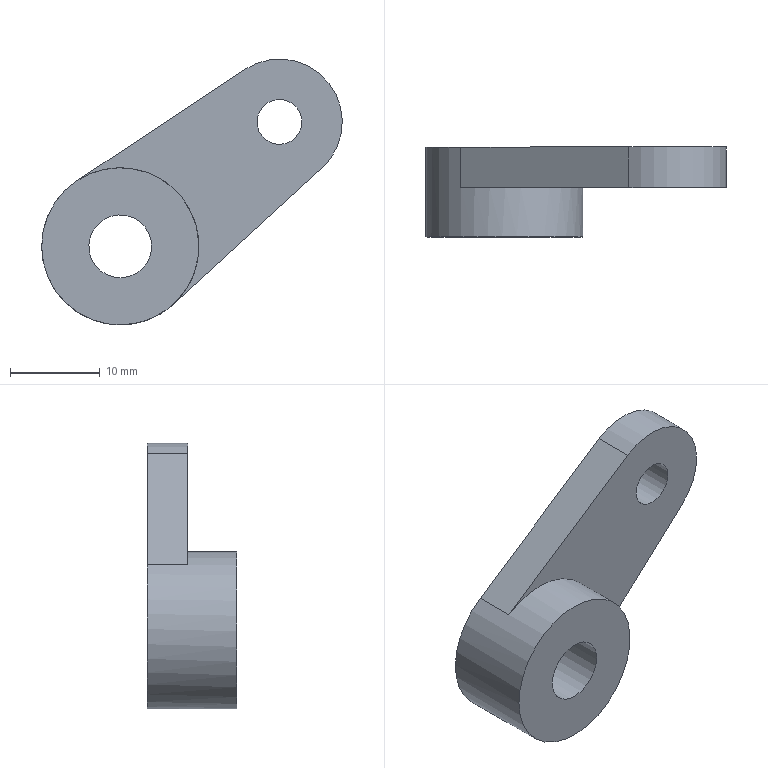Component | NX | 9 | 1 solid | 9 faces | box 33.48 x 10 x 29.6 mm | volume 3337 mm3 | plane 5 | cylinder 4 | commonest cylinder face diameters 14 x1 5 x1 17.5 x1 7 x1
STEP:
#1=CARTESIAN_POINT('',(0.,0.,0.));
#2=DIRECTION('',(0.,0.,1.));
#3=DIRECTION('',(1.,0.,0.));
#4=AXIS2_PLACEMENT_3D('',#1,#2,#3);
#5=CARTESIAN_POINT('',(-294.831,190.749,-231.716));
#6=VERTEX_POINT('',#5);
#7=CARTESIAN_POINT('',(-278.282,190.749,-216.572));
#8=VERTEX_POINT('',#7);
#9=CARTESIAN_POINT('',(-294.831,190.749,-231.716));
#10=DIRECTION('',(0.7377,0.,0.6751));
#11=VECTOR('',#10,1.);
#12=LINE('',#9,#11);
#13=CARTESIAN_POINT('',(-294.831,186.249,-231.716));
#14=DIRECTION('',(-0.6751,0.,0.7377));
#15=DIRECTION('',(-0.7377,0.,-0.6751));
#16=AXIS2_PLACEMENT_3D('',#13,#14,#15);
#17=PLANE('',#16);
#18=CARTESIAN_POINT('',(0.,-4.5));
#19=DIRECTION('',(-1.,0.));
#20=VECTOR('',#19,1.);
#21=LINE('',#18,#20);
#22=(GEOMETRIC_REPRESENTATION_CONTEXT(2)PARAMETRIC_REPRESENTATION_CONTEXT()REPRESENTATION_CONTEXT('',''));
#23=DEFINITIONAL_REPRESENTATION('',(#21),#22);
#24=PCURVE('',#17,#23);
#25=CARTESIAN_POINT('',(-300.738,190.749,-225.261));
#26=DIRECTION('',(0.,1.,0.));
#27=DIRECTION('',(-0.788,0.,-0.6157));
#28=AXIS2_PLACEMENT_3D('',#25,#26,#27);
#29=PLANE('',#28);
#30=CARTESIAN_POINT('',(-0.6806,-8.723));
#31=DIRECTION('',(-0.997,0.07778));
#32=VECTOR('',#31,1.);
#33=LINE('',#30,#32);
#34=(GEOMETRIC_REPRESENTATION_CONTEXT(2)PARAMETRIC_REPRESENTATION_CONTEXT()REPRESENTATION_CONTEXT('',''));
#35=DEFINITIONAL_REPRESENTATION('',(#33),#34);
#36=PCURVE('',#29,#35);
#37=SURFACE_CURVE('',#12,(#24,#36),.PCURVE_S1.);
#38=EDGE_CURVE('',#6,#8,#37,.T.);
#39=ORIENTED_EDGE('',*,*,#38,.T.);
#40=CARTESIAN_POINT('',(-278.282,186.249,-216.572));
#41=VERTEX_POINT('',#40);
#42=CARTESIAN_POINT('',(-278.282,186.249,-216.572));
#43=DIRECTION('',(0.,1.,0.));
#44=VECTOR('',#43,1.);
#45=LINE('',#42,#44);
#46=CARTESIAN_POINT('',(-22.432,0.));
#47=DIRECTION('',(0.,-1.));
#48=VECTOR('',#47,1.);
#49=LINE('',#46,#48);
#50=(GEOMETRIC_REPRESENTATION_CONTEXT(2)PARAMETRIC_REPRESENTATION_CONTEXT()REPRESENTATION_CONTEXT('',''));
#51=DEFINITIONAL_REPRESENTATION('',(#49),#50);
#52=PCURVE('',#17,#51);
#53=CARTESIAN_POINT('',(-283.008,186.249,-211.408));
#54=DIRECTION('',(0.,1.,0.));
#55=DIRECTION('',(-0.788,0.,-0.6157));
#56=AXIS2_PLACEMENT_3D('',#53,#54,#55);
#57=CYLINDRICAL_SURFACE('',#56,7.);
#58=CARTESIAN_POINT('',(4.635,0.));
#59=DIRECTION('',(0.,1.));
#60=VECTOR('',#59,1.);
#61=LINE('',#58,#60);
#62=(GEOMETRIC_REPRESENTATION_CONTEXT(2)PARAMETRIC_REPRESENTATION_CONTEXT()REPRESENTATION_CONTEXT('',''));
#63=DEFINITIONAL_REPRESENTATION('',(#61),#62);
#64=PCURVE('',#57,#63);
#65=SURFACE_CURVE('',#45,(#52,#64),.PCURVE_S1.);
#66=EDGE_CURVE('',#41,#8,#65,.T.);
#67=ORIENTED_EDGE('',*,*,#66,.F.);
#68=CARTESIAN_POINT('',(-294.831,186.249,-231.716));
#69=VERTEX_POINT('',#68);
#70=CARTESIAN_POINT('',(-294.831,186.249,-231.716));
#71=DIRECTION('',(0.7377,0.,0.6751));
#72=VECTOR('',#71,1.);
#73=LINE('',#70,#72);
#74=CARTESIAN_POINT('',(0.,0.));
#75=DIRECTION('',(-1.,0.));
#76=VECTOR('',#75,1.);
#77=LINE('',#74,#76);
#78=(GEOMETRIC_REPRESENTATION_CONTEXT(2)PARAMETRIC_REPRESENTATION_CONTEXT()REPRESENTATION_CONTEXT('',''));
#79=DEFINITIONAL_REPRESENTATION('',(#77),#78);
#80=PCURVE('',#17,#79);
#81=CARTESIAN_POINT('',(-300.738,186.249,-225.261));
#82=DIRECTION('',(0.,1.,0.));
#83=DIRECTION('',(-0.788,0.,-0.6157));
#84=AXIS2_PLACEMENT_3D('',#81,#82,#83);
#85=PLANE('',#84);
#86=CARTESIAN_POINT('',(-0.6806,-8.723));
#87=DIRECTION('',(-0.997,0.07778));
#88=VECTOR('',#87,1.);
#89=LINE('',#86,#88);
#90=(GEOMETRIC_REPRESENTATION_CONTEXT(2)PARAMETRIC_REPRESENTATION_CONTEXT()REPRESENTATION_CONTEXT('',''));
#91=DEFINITIONAL_REPRESENTATION('',(#89),#90);
#92=PCURVE('',#85,#91);
#93=SURFACE_CURVE('',#73,(#80,#92),.PCURVE_S1.);
#94=EDGE_CURVE('',#69,#41,#93,.T.);
#95=ORIENTED_EDGE('',*,*,#94,.F.);
#96=CARTESIAN_POINT('',(-294.831,186.249,-231.716));
#97=DIRECTION('',(0.,1.,0.));
#98=VECTOR('',#97,1.);
#99=LINE('',#96,#98);
#100=CARTESIAN_POINT('',(0.,0.));
#101=DIRECTION('',(0.,-1.));
#102=VECTOR('',#101,1.);
#103=LINE('',#100,#102);
#104=(GEOMETRIC_REPRESENTATION_CONTEXT(2)PARAMETRIC_REPRESENTATION_CONTEXT()REPRESENTATION_CONTEXT('',''));
#105=DEFINITIONAL_REPRESENTATION('',(#103),#104);
#106=PCURVE('',#17,#105);
#107=CARTESIAN_POINT('',(-300.738,180.749,-225.261));
#108=DIRECTION('',(0.,1.,0.));
#109=DIRECTION('',(-0.788,0.,-0.6157));
#110=AXIS2_PLACEMENT_3D('',#107,#108,#109);
#111=CYLINDRICAL_SURFACE('',#110,8.75);
#112=CARTESIAN_POINT('',(4.635,5.5));
#113=DIRECTION('',(0.,1.));
#114=VECTOR('',#113,1.);
#115=LINE('',#112,#114);
#116=(GEOMETRIC_REPRESENTATION_CONTEXT(2)PARAMETRIC_REPRESENTATION_CONTEXT()REPRESENTATION_CONTEXT('',''));
#117=DEFINITIONAL_REPRESENTATION('',(#115),#116);
#118=PCURVE('',#111,#117);
#119=SURFACE_CURVE('',#99,(#106,#118),.PCURVE_S1.);
#120=EDGE_CURVE('',#69,#6,#119,.T.);
#121=ORIENTED_EDGE('',*,*,#120,.T.);
#122=EDGE_LOOP('',(#39,#67,#95,#121));
#123=FACE_BOUND('',#122,.T.);
#124=ADVANCED_FACE('',(#123),#17,.F.);
#125=CARTESIAN_POINT('',(-286.875,190.749,-205.574));
#126=VERTEX_POINT('',#125);
#127=CARTESIAN_POINT('',(-283.008,190.749,-211.408));
#128=DIRECTION('',(0.,-1.,0.));
#129=DIRECTION('',(0.788,0.,0.6157));
#130=AXIS2_PLACEMENT_3D('',#127,#128,#129);
#131=CIRCLE('',#130,7.);
#132=CARTESIAN_POINT('',(9.425,4.5));
#133=DIRECTION('',(-1.,0.));
#134=VECTOR('',#133,1.);
#135=LINE('',#132,#134);
#136=(GEOMETRIC_REPRESENTATION_CONTEXT(2)PARAMETRIC_REPRESENTATION_CONTEXT()REPRESENTATION_CONTEXT('',''));
#137=DEFINITIONAL_REPRESENTATION('',(#135),#136);
#138=PCURVE('',#57,#137);
#139=CARTESIAN_POINT('',(-29.5,-0.));
#140=CARTESIAN_POINT('',(-29.5,12.124));
#141=CARTESIAN_POINT('',(-19.,6.062));
#142=CARTESIAN_POINT('',(-8.5,-0.));
#143=CARTESIAN_POINT('',(-19.,-6.062));
#144=CARTESIAN_POINT('',(-29.5,-12.124));
#145=CARTESIAN_POINT('',(-29.5,-0.));
#146=(BOUNDED_CURVE()B_SPLINE_CURVE(2,(#139,#140,#141,#142,#143,#144,#145),.UNSPECIFIED.,.T.,.F.)B_SPLINE_CURVE_WITH_KNOTS((1,2,2,2,2,1),(-2.094,0.,2.094,4.189,6.283,8.378),.UNSPECIFIED.)CURVE()GEOMETRIC_REPRESENTATION_ITEM()RATIONAL_B_SPLINE_CURVE((1.,0.5,1.,0.5,1.,0.5,1.))REPRESENTATION_ITEM(''));
#147=(GEOMETRIC_REPRESENTATION_CONTEXT(2)PARAMETRIC_REPRESENTATION_CONTEXT()REPRESENTATION_CONTEXT('',''));
#148=DEFINITIONAL_REPRESENTATION('',(#146),#147);
#149=PCURVE('',#29,#148);
#150=SURFACE_CURVE('',#131,(#138,#149),.PCURVE_S1.);
#151=EDGE_CURVE('',#8,#126,#150,.T.);
#152=ORIENTED_EDGE('',*,*,#151,.T.);
#153=CARTESIAN_POINT('',(-286.875,186.249,-205.574));
#154=VERTEX_POINT('',#153);
#155=CARTESIAN_POINT('',(-286.875,186.249,-205.574));
#156=DIRECTION('',(0.,1.,0.));
#157=VECTOR('',#156,1.);
#158=LINE('',#155,#157);
#159=CARTESIAN_POINT('',(1.649,0.));
#160=DIRECTION('',(0.,1.));
#161=VECTOR('',#160,1.);
#162=LINE('',#159,#161);
#163=(GEOMETRIC_REPRESENTATION_CONTEXT(2)PARAMETRIC_REPRESENTATION_CONTEXT()REPRESENTATION_CONTEXT('',''));
#164=DEFINITIONAL_REPRESENTATION('',(#162),#163);
#165=PCURVE('',#57,#164);
#166=CARTESIAN_POINT('',(-286.875,186.249,-205.574));
#167=DIRECTION('',(0.5525,0.,-0.8335));
#168=DIRECTION('',(0.8335,0.,0.5525));
#169=AXIS2_PLACEMENT_3D('',#166,#167,#168);
#170=PLANE('',#169);
#171=CARTESIAN_POINT('',(0.,0.));
#172=DIRECTION('',(0.,-1.));
#173=VECTOR('',#172,1.);
#174=LINE('',#171,#173);
#175=(GEOMETRIC_REPRESENTATION_CONTEXT(2)PARAMETRIC_REPRESENTATION_CONTEXT()REPRESENTATION_CONTEXT('',''));
#176=DEFINITIONAL_REPRESENTATION('',(#174),#175);
#177=PCURVE('',#170,#176);
#178=SURFACE_CURVE('',#158,(#165,#177),.PCURVE_S1.);
#179=EDGE_CURVE('',#154,#126,#178,.T.);
#180=ORIENTED_EDGE('',*,*,#179,.F.);
#181=CARTESIAN_POINT('',(-283.008,186.249,-211.408));
#182=DIRECTION('',(0.,-1.,0.));
#183=DIRECTION('',(0.788,0.,0.6157));
#184=AXIS2_PLACEMENT_3D('',#181,#182,#183);
#185=CIRCLE('',#184,7.);
#186=CARTESIAN_POINT('',(9.425,0.));
#187=DIRECTION('',(-1.,0.));
#188=VECTOR('',#187,1.);
#189=LINE('',#186,#188);
#190=(GEOMETRIC_REPRESENTATION_CONTEXT(2)PARAMETRIC_REPRESENTATION_CONTEXT()REPRESENTATION_CONTEXT('',''));
#191=DEFINITIONAL_REPRESENTATION('',(#189),#190);
#192=PCURVE('',#57,#191);
#193=CARTESIAN_POINT('',(-29.5,-0.));
#194=CARTESIAN_POINT('',(-29.5,12.124));
#195=CARTESIAN_POINT('',(-19.,6.062));
#196=CARTESIAN_POINT('',(-8.5,-0.));
#197=CARTESIAN_POINT('',(-19.,-6.062));
#198=CARTESIAN_POINT('',(-29.5,-12.124));
#199=CARTESIAN_POINT('',(-29.5,-0.));
#200=(BOUNDED_CURVE()B_SPLINE_CURVE(2,(#193,#194,#195,#196,#197,#198,#199),.UNSPECIFIED.,.T.,.F.)B_SPLINE_CURVE_WITH_KNOTS((1,2,2,2,2,1),(-2.094,0.,2.094,4.189,6.283,8.378),.UNSPECIFIED.)CURVE()GEOMETRIC_REPRESENTATION_ITEM()RATIONAL_B_SPLINE_CURVE((1.,0.5,1.,0.5,1.,0.5,1.))REPRESENTATION_ITEM(''));
#201=(GEOMETRIC_REPRESENTATION_CONTEXT(2)PARAMETRIC_REPRESENTATION_CONTEXT()REPRESENTATION_CONTEXT('',''));
#202=DEFINITIONAL_REPRESENTATION('',(#200),#201);
#203=PCURVE('',#85,#202);
#204=SURFACE_CURVE('',#185,(#192,#203),.PCURVE_S1.);
#205=EDGE_CURVE('',#41,#154,#204,.T.);
#206=ORIENTED_EDGE('',*,*,#205,.F.);
#207=ORIENTED_EDGE('',*,*,#66,.T.);
#208=EDGE_LOOP('',(#152,#180,#206,#207));
#209=FACE_BOUND('',#208,.T.);
#210=ADVANCED_FACE('',(#209),#57,.T.);
#211=CARTESIAN_POINT('',(-305.572,190.749,-217.967));
#212=VERTEX_POINT('',#211);
#213=CARTESIAN_POINT('',(-286.875,190.749,-205.574));
#214=DIRECTION('',(-0.8335,0.,-0.5525));
#215=VECTOR('',#214,1.);
#216=LINE('',#213,#215);
#217=CARTESIAN_POINT('',(0.,-4.5));
#218=DIRECTION('',(-1.,0.));
#219=VECTOR('',#218,1.);
#220=LINE('',#217,#219);
#221=(GEOMETRIC_REPRESENTATION_CONTEXT(2)PARAMETRIC_REPRESENTATION_CONTEXT()REPRESENTATION_CONTEXT('',''));
#222=DEFINITIONAL_REPRESENTATION('',(#220),#221);
#223=PCURVE('',#170,#222);
#224=CARTESIAN_POINT('',(-23.044,6.979));
#225=DIRECTION('',(0.997,0.07778));
#226=VECTOR('',#225,1.);
#227=LINE('',#224,#226);
#228=(GEOMETRIC_REPRESENTATION_CONTEXT(2)PARAMETRIC_REPRESENTATION_CONTEXT()REPRESENTATION_CONTEXT('',''));
#229=DEFINITIONAL_REPRESENTATION('',(#227),#228);
#230=PCURVE('',#29,#229);
#231=SURFACE_CURVE('',#216,(#223,#230),.PCURVE_S1.);
#232=EDGE_CURVE('',#126,#212,#231,.T.);
#233=ORIENTED_EDGE('',*,*,#232,.T.);
#234=CARTESIAN_POINT('',(-305.572,186.249,-217.967));
#235=VERTEX_POINT('',#234);
#236=CARTESIAN_POINT('',(-305.572,186.249,-217.967));
#237=DIRECTION('',(0.,1.,0.));
#238=VECTOR('',#237,1.);
#239=LINE('',#236,#238);
#240=CARTESIAN_POINT('',(-22.432,0.));
#241=DIRECTION('',(0.,-1.));
#242=VECTOR('',#241,1.);
#243=LINE('',#240,#242);
#244=(GEOMETRIC_REPRESENTATION_CONTEXT(2)PARAMETRIC_REPRESENTATION_CONTEXT()REPRESENTATION_CONTEXT('',''));
#245=DEFINITIONAL_REPRESENTATION('',(#243),#244);
#246=PCURVE('',#170,#245);
#247=CARTESIAN_POINT('',(7.932,5.5));
#248=DIRECTION('',(0.,1.));
#249=VECTOR('',#248,1.);
#250=LINE('',#247,#249);
#251=(GEOMETRIC_REPRESENTATION_CONTEXT(2)PARAMETRIC_REPRESENTATION_CONTEXT()REPRESENTATION_CONTEXT('',''));
#252=DEFINITIONAL_REPRESENTATION('',(#250),#251);
#253=PCURVE('',#111,#252);
#254=SURFACE_CURVE('',#239,(#246,#253),.PCURVE_S1.);
#255=EDGE_CURVE('',#235,#212,#254,.T.);
#256=ORIENTED_EDGE('',*,*,#255,.F.);
#257=CARTESIAN_POINT('',(-286.875,186.249,-205.574));
#258=DIRECTION('',(-0.8335,0.,-0.5525));
#259=VECTOR('',#258,1.);
#260=LINE('',#257,#259);
#261=CARTESIAN_POINT('',(0.,0.));
#262=DIRECTION('',(-1.,0.));
#263=VECTOR('',#262,1.);
#264=LINE('',#261,#263);
#265=(GEOMETRIC_REPRESENTATION_CONTEXT(2)PARAMETRIC_REPRESENTATION_CONTEXT()REPRESENTATION_CONTEXT('',''));
#266=DEFINITIONAL_REPRESENTATION('',(#264),#265);
#267=PCURVE('',#170,#266);
#268=CARTESIAN_POINT('',(-23.044,6.979));
#269=DIRECTION('',(0.997,0.07778));
#270=VECTOR('',#269,1.);
#271=LINE('',#268,#270);
#272=(GEOMETRIC_REPRESENTATION_CONTEXT(2)PARAMETRIC_REPRESENTATION_CONTEXT()REPRESENTATION_CONTEXT('',''));
#273=DEFINITIONAL_REPRESENTATION('',(#271),#272);
#274=PCURVE('',#85,#273);
#275=SURFACE_CURVE('',#260,(#267,#274),.PCURVE_S1.);
#276=EDGE_CURVE('',#154,#235,#275,.T.);
#277=ORIENTED_EDGE('',*,*,#276,.F.);
#278=ORIENTED_EDGE('',*,*,#179,.T.);
#279=EDGE_LOOP('',(#233,#256,#277,#278));
#280=FACE_BOUND('',#279,.T.);
#281=ADVANCED_FACE('',(#280),#170,.F.);
#282=CARTESIAN_POINT('',(-281.038,186.249,-209.869));
#283=VERTEX_POINT('',#282);
#284=CARTESIAN_POINT('',(-283.008,186.249,-211.408));
#285=DIRECTION('',(0.,-1.,0.));
#286=DIRECTION('',(0.788,0.,0.6157));
#287=AXIS2_PLACEMENT_3D('',#284,#285,#286);
#288=CIRCLE('',#287,2.5);
#289=CARTESIAN_POINT('',(-283.008,186.249,-211.408));
#290=DIRECTION('',(0.,1.,0.));
#291=DIRECTION('',(-0.788,0.,-0.6157));
#292=AXIS2_PLACEMENT_3D('',#289,#290,#291);
#293=CYLINDRICAL_SURFACE('',#292,2.5);
#294=CARTESIAN_POINT('',(9.425,0.));
#295=DIRECTION('',(-1.,0.));
#296=VECTOR('',#295,1.);
#297=LINE('',#294,#296);
#298=(GEOMETRIC_REPRESENTATION_CONTEXT(2)PARAMETRIC_REPRESENTATION_CONTEXT()REPRESENTATION_CONTEXT('',''));
#299=DEFINITIONAL_REPRESENTATION('',(#297),#298);
#300=PCURVE('',#293,#299);
#301=CARTESIAN_POINT('',(-25.,-0.));
#302=CARTESIAN_POINT('',(-25.,4.33));
#303=CARTESIAN_POINT('',(-21.25,2.165));
#304=CARTESIAN_POINT('',(-17.5,-0.));
#305=CARTESIAN_POINT('',(-21.25,-2.165));
#306=CARTESIAN_POINT('',(-25.,-4.33));
#307=CARTESIAN_POINT('',(-25.,-0.));
#308=(BOUNDED_CURVE()B_SPLINE_CURVE(2,(#301,#302,#303,#304,#305,#306,#307),.UNSPECIFIED.,.T.,.F.)B_SPLINE_CURVE_WITH_KNOTS((1,2,2,2,2,1),(-2.094,0.,2.094,4.189,6.283,8.378),.UNSPECIFIED.)CURVE()GEOMETRIC_REPRESENTATION_ITEM()RATIONAL_B_SPLINE_CURVE((1.,0.5,1.,0.5,1.,0.5,1.))REPRESENTATION_ITEM(''));
#309=(GEOMETRIC_REPRESENTATION_CONTEXT(2)PARAMETRIC_REPRESENTATION_CONTEXT()REPRESENTATION_CONTEXT('',''));
#310=DEFINITIONAL_REPRESENTATION('',(#308),#309);
#311=PCURVE('',#85,#310);
#312=SURFACE_CURVE('',#288,(#300,#311),.PCURVE_S1.);
#313=EDGE_CURVE('',#283,#283,#312,.T.);
#314=ORIENTED_EDGE('',*,*,#313,.F.);
#315=CARTESIAN_POINT('',(-281.038,190.749,-209.869));
#316=VERTEX_POINT('',#315);
#317=CARTESIAN_POINT('',(-281.038,186.249,-209.869));
#318=CARTESIAN_POINT('',(-281.038,190.749,-209.869));
#319=B_SPLINE_CURVE_WITH_KNOTS('',1,(#317,#318),.UNSPECIFIED.,.F.,.F.,(2,2),(0.,4.5),.PIECEWISE_BEZIER_KNOTS.);
#320=CARTESIAN_POINT('',(9.425,0.));
#321=DIRECTION('',(0.,1.));
#322=VECTOR('',#321,1.);
#323=LINE('',#320,#322);
#324=(GEOMETRIC_REPRESENTATION_CONTEXT(2)PARAMETRIC_REPRESENTATION_CONTEXT()REPRESENTATION_CONTEXT('',''));
#325=DEFINITIONAL_REPRESENTATION('',(#323),#324);
#326=PCURVE('',#293,#325);
#327=CARTESIAN_POINT('',(3.142,0.));
#328=DIRECTION('',(0.,1.));
#329=VECTOR('',#328,1.);
#330=LINE('',#327,#329);
#331=(GEOMETRIC_REPRESENTATION_CONTEXT(2)PARAMETRIC_REPRESENTATION_CONTEXT()REPRESENTATION_CONTEXT('',''));
#332=DEFINITIONAL_REPRESENTATION('',(#330),#331);
#333=PCURVE('',#293,#332);
#334=SEAM_CURVE('',#319,(#326,#333),.PCURVE_S1.);
#335=EDGE_CURVE('',#283,#316,#334,.T.);
#336=ORIENTED_EDGE('',*,*,#335,.T.);
#337=CARTESIAN_POINT('',(-283.008,190.749,-211.408));
#338=DIRECTION('',(0.,-1.,0.));
#339=DIRECTION('',(0.788,0.,0.6157));
#340=AXIS2_PLACEMENT_3D('',#337,#338,#339);
#341=CIRCLE('',#340,2.5);
#342=CARTESIAN_POINT('',(9.425,4.5));
#343=DIRECTION('',(-1.,0.));
#344=VECTOR('',#343,1.);
#345=LINE('',#342,#344);
#346=(GEOMETRIC_REPRESENTATION_CONTEXT(2)PARAMETRIC_REPRESENTATION_CONTEXT()REPRESENTATION_CONTEXT('',''));
#347=DEFINITIONAL_REPRESENTATION('',(#345),#346);
#348=PCURVE('',#293,#347);
#349=CARTESIAN_POINT('',(-25.,-0.));
#350=CARTESIAN_POINT('',(-25.,4.33));
#351=CARTESIAN_POINT('',(-21.25,2.165));
#352=CARTESIAN_POINT('',(-17.5,-0.));
#353=CARTESIAN_POINT('',(-21.25,-2.165));
#354=CARTESIAN_POINT('',(-25.,-4.33));
#355=CARTESIAN_POINT('',(-25.,-0.));
#356=(BOUNDED_CURVE()B_SPLINE_CURVE(2,(#349,#350,#351,#352,#353,#354,#355),.UNSPECIFIED.,.T.,.F.)B_SPLINE_CURVE_WITH_KNOTS((1,2,2,2,2,1),(-2.094,0.,2.094,4.189,6.283,8.378),.UNSPECIFIED.)CURVE()GEOMETRIC_REPRESENTATION_ITEM()RATIONAL_B_SPLINE_CURVE((1.,0.5,1.,0.5,1.,0.5,1.))REPRESENTATION_ITEM(''));
#357=(GEOMETRIC_REPRESENTATION_CONTEXT(2)PARAMETRIC_REPRESENTATION_CONTEXT()REPRESENTATION_CONTEXT('',''));
#358=DEFINITIONAL_REPRESENTATION('',(#356),#357);
#359=PCURVE('',#29,#358);
#360=SURFACE_CURVE('',#341,(#348,#359),.PCURVE_S1.);
#361=EDGE_CURVE('',#316,#316,#360,.T.);
#362=ORIENTED_EDGE('',*,*,#361,.T.);
#363=ORIENTED_EDGE('',*,*,#335,.F.);
#364=EDGE_LOOP('',(#314,#336,#362,#363));
#365=FACE_BOUND('',#364,.F.);
#366=ADVANCED_FACE('',(#365),#293,.F.);
#367=CARTESIAN_POINT('',(-300.738,186.249,-225.261));
#368=DIRECTION('',(0.,1.,0.));
#369=DIRECTION('',(0.788,0.,0.6157));
#370=AXIS2_PLACEMENT_3D('',#367,#368,#369);
#371=CIRCLE('',#370,8.75);
#372=CARTESIAN_POINT('',(0.,0.));
#373=DIRECTION('',(-1.,-0.));
#374=AXIS2_PLACEMENT_2D('',#372,#373);
#375=CIRCLE('',#374,8.75);
#376=(GEOMETRIC_REPRESENTATION_CONTEXT(2)PARAMETRIC_REPRESENTATION_CONTEXT()REPRESENTATION_CONTEXT('',''));
#377=DEFINITIONAL_REPRESENTATION('',(#375),#376);
#378=PCURVE('',#85,#377);
#379=CARTESIAN_POINT('',(-3.142,5.5));
#380=DIRECTION('',(1.,0.));
#381=VECTOR('',#380,1.);
#382=LINE('',#379,#381);
#383=(GEOMETRIC_REPRESENTATION_CONTEXT(2)PARAMETRIC_REPRESENTATION_CONTEXT()REPRESENTATION_CONTEXT('',''));
#384=DEFINITIONAL_REPRESENTATION('',(#382),#383);
#385=PCURVE('',#111,#384);
#386=SURFACE_CURVE('',#371,(#378,#385),.PCURVE_S1.);
#387=EDGE_CURVE('',#235,#69,#386,.T.);
#388=ORIENTED_EDGE('',*,*,#387,.T.);
#389=ORIENTED_EDGE('',*,*,#94,.T.);
#390=ORIENTED_EDGE('',*,*,#205,.T.);
#391=ORIENTED_EDGE('',*,*,#276,.T.);
#392=EDGE_LOOP('',(#388,#389,#390,#391));
#393=FACE_BOUND('',#392,.T.);
#394=ORIENTED_EDGE('',*,*,#313,.F.);
#395=EDGE_LOOP('',(#394));
#396=FACE_BOUND('',#395,.T.);
#397=ADVANCED_FACE('',(#393,#396),#85,.F.);
#398=ORIENTED_EDGE('',*,*,#38,.F.);
#399=CARTESIAN_POINT('',(-300.738,190.749,-225.261));
#400=DIRECTION('',(0.,-1.,0.));
#401=DIRECTION('',(0.788,0.,0.6157));
#402=AXIS2_PLACEMENT_3D('',#399,#400,#401);
#403=CIRCLE('',#402,8.75);
#404=CARTESIAN_POINT('',(-8.75,-0.));
#405=CARTESIAN_POINT('',(-8.75,15.155));
#406=CARTESIAN_POINT('',(4.375,7.578));
#407=CARTESIAN_POINT('',(17.5,0.));
#408=CARTESIAN_POINT('',(4.375,-7.578));
#409=CARTESIAN_POINT('',(-8.75,-15.155));
#410=CARTESIAN_POINT('',(-8.75,-0.));
#411=(BOUNDED_CURVE()B_SPLINE_CURVE(2,(#404,#405,#406,#407,#408,#409,#410),.UNSPECIFIED.,.T.,.F.)B_SPLINE_CURVE_WITH_KNOTS((1,2,2,2,2,1),(-2.094,0.,2.094,4.189,6.283,8.378),.UNSPECIFIED.)CURVE()GEOMETRIC_REPRESENTATION_ITEM()RATIONAL_B_SPLINE_CURVE((1.,0.5,1.,0.5,1.,0.5,1.))REPRESENTATION_ITEM(''));
#412=(GEOMETRIC_REPRESENTATION_CONTEXT(2)PARAMETRIC_REPRESENTATION_CONTEXT()REPRESENTATION_CONTEXT('',''));
#413=DEFINITIONAL_REPRESENTATION('',(#411),#412);
#414=PCURVE('',#29,#413);
#415=CARTESIAN_POINT('',(9.425,10.));
#416=DIRECTION('',(-1.,0.));
#417=VECTOR('',#416,1.);
#418=LINE('',#415,#417);
#419=(GEOMETRIC_REPRESENTATION_CONTEXT(2)PARAMETRIC_REPRESENTATION_CONTEXT()REPRESENTATION_CONTEXT('',''));
#420=DEFINITIONAL_REPRESENTATION('',(#418),#419);
#421=PCURVE('',#111,#420);
#422=SURFACE_CURVE('',#403,(#414,#421),.PCURVE_S1.);
#423=EDGE_CURVE('',#212,#6,#422,.T.);
#424=ORIENTED_EDGE('',*,*,#423,.F.);
#425=ORIENTED_EDGE('',*,*,#232,.F.);
#426=ORIENTED_EDGE('',*,*,#151,.F.);
#427=EDGE_LOOP('',(#398,#424,#425,#426));
#428=FACE_BOUND('',#427,.T.);
#429=ORIENTED_EDGE('',*,*,#361,.T.);
#430=EDGE_LOOP('',(#429));
#431=FACE_BOUND('',#430,.T.);
#432=CARTESIAN_POINT('',(-297.98,190.749,-223.106));
#433=VERTEX_POINT('',#432);
#434=CARTESIAN_POINT('',(-300.738,190.749,-225.261));
#435=DIRECTION('',(0.,-1.,0.));
#436=DIRECTION('',(0.788,0.,0.6157));
#437=AXIS2_PLACEMENT_3D('',#434,#435,#436);
#438=CIRCLE('',#437,3.5);
#439=CARTESIAN_POINT('',(-3.5,-0.));
#440=CARTESIAN_POINT('',(-3.5,6.062));
#441=CARTESIAN_POINT('',(1.75,3.031));
#442=CARTESIAN_POINT('',(7.,0.));
#443=CARTESIAN_POINT('',(1.75,-3.031));
#444=CARTESIAN_POINT('',(-3.5,-6.062));
#445=CARTESIAN_POINT('',(-3.5,-0.));
#446=(BOUNDED_CURVE()B_SPLINE_CURVE(2,(#439,#440,#441,#442,#443,#444,#445),.UNSPECIFIED.,.T.,.F.)B_SPLINE_CURVE_WITH_KNOTS((1,2,2,2,2,1),(-2.094,0.,2.094,4.189,6.283,8.378),.UNSPECIFIED.)CURVE()GEOMETRIC_REPRESENTATION_ITEM()RATIONAL_B_SPLINE_CURVE((1.,0.5,1.,0.5,1.,0.5,1.))REPRESENTATION_ITEM(''));
#447=(GEOMETRIC_REPRESENTATION_CONTEXT(2)PARAMETRIC_REPRESENTATION_CONTEXT()REPRESENTATION_CONTEXT('',''));
#448=DEFINITIONAL_REPRESENTATION('',(#446),#447);
#449=PCURVE('',#29,#448);
#450=CARTESIAN_POINT('',(-300.738,180.749,-225.261));
#451=DIRECTION('',(0.,1.,0.));
#452=DIRECTION('',(-0.788,0.,-0.6157));
#453=AXIS2_PLACEMENT_3D('',#450,#451,#452);
#454=CYLINDRICAL_SURFACE('',#453,3.5);
#455=CARTESIAN_POINT('',(9.425,10.));
#456=DIRECTION('',(-1.,0.));
#457=VECTOR('',#456,1.);
#458=LINE('',#455,#457);
#459=(GEOMETRIC_REPRESENTATION_CONTEXT(2)PARAMETRIC_REPRESENTATION_CONTEXT()REPRESENTATION_CONTEXT('',''));
#460=DEFINITIONAL_REPRESENTATION('',(#458),#459);
#461=PCURVE('',#454,#460);
#462=SURFACE_CURVE('',#438,(#449,#461),.PCURVE_S1.);
#463=EDGE_CURVE('',#433,#433,#462,.T.);
#464=ORIENTED_EDGE('',*,*,#463,.T.);
#465=EDGE_LOOP('',(#464));
#466=FACE_BOUND('',#465,.T.);
#467=ADVANCED_FACE('',(#428,#431,#466),#29,.T.);
#468=ORIENTED_EDGE('',*,*,#120,.F.);
#469=ORIENTED_EDGE('',*,*,#387,.F.);
#470=CARTESIAN_POINT('',(-305.572,180.749,-217.967));
#471=VERTEX_POINT('',#470);
#472=CARTESIAN_POINT('',(-305.572,180.749,-217.967));
#473=CARTESIAN_POINT('',(-305.572,186.249,-217.967));
#474=B_SPLINE_CURVE_WITH_KNOTS('',1,(#472,#473),.UNSPECIFIED.,.F.,.F.,(2,2),(0.,5.5),.PIECEWISE_BEZIER_KNOTS.);
#475=CARTESIAN_POINT('',(1.649,0.));
#476=DIRECTION('',(0.,1.));
#477=VECTOR('',#476,1.);
#478=LINE('',#475,#477);
#479=(GEOMETRIC_REPRESENTATION_CONTEXT(2)PARAMETRIC_REPRESENTATION_CONTEXT()REPRESENTATION_CONTEXT('',''));
#480=DEFINITIONAL_REPRESENTATION('',(#478),#479);
#481=PCURVE('',#111,#480);
#482=CARTESIAN_POINT('',(7.932,0.));
#483=DIRECTION('',(0.,1.));
#484=VECTOR('',#483,1.);
#485=LINE('',#482,#484);
#486=(GEOMETRIC_REPRESENTATION_CONTEXT(2)PARAMETRIC_REPRESENTATION_CONTEXT()REPRESENTATION_CONTEXT('',''));
#487=DEFINITIONAL_REPRESENTATION('',(#485),#486);
#488=PCURVE('',#111,#487);
#489=SEAM_CURVE('',#474,(#481,#488),.PCURVE_S1.);
#490=EDGE_CURVE('',#471,#235,#489,.T.);
#491=ORIENTED_EDGE('',*,*,#490,.F.);
#492=CARTESIAN_POINT('',(-293.843,180.749,-219.873));
#493=VERTEX_POINT('',#492);
#494=CARTESIAN_POINT('',(-300.738,180.749,-225.261));
#495=DIRECTION('',(0.,-1.,0.));
#496=DIRECTION('',(0.788,0.,0.6157));
#497=AXIS2_PLACEMENT_3D('',#494,#495,#496);
#498=CIRCLE('',#497,8.75);
#499=CARTESIAN_POINT('',(3.142,0.));
#500=DIRECTION('',(-1.,0.));
#501=VECTOR('',#500,1.);
#502=LINE('',#499,#501);
#503=(GEOMETRIC_REPRESENTATION_CONTEXT(2)PARAMETRIC_REPRESENTATION_CONTEXT()REPRESENTATION_CONTEXT('',''));
#504=DEFINITIONAL_REPRESENTATION('',(#502),#503);
#505=PCURVE('',#111,#504);
#506=CARTESIAN_POINT('',(-300.738,180.749,-225.261));
#507=DIRECTION('',(0.,-1.,0.));
#508=DIRECTION('',(0.788,0.,0.6157));
#509=AXIS2_PLACEMENT_3D('',#506,#507,#508);
#510=PLANE('',#509);
#511=CARTESIAN_POINT('',(0.,0.));
#512=DIRECTION('',(1.,-0.));
#513=AXIS2_PLACEMENT_2D('',#511,#512);
#514=CIRCLE('',#513,8.75);
#515=(GEOMETRIC_REPRESENTATION_CONTEXT(2)PARAMETRIC_REPRESENTATION_CONTEXT()REPRESENTATION_CONTEXT('',''));
#516=DEFINITIONAL_REPRESENTATION('',(#514),#515);
#517=PCURVE('',#510,#516);
#518=SURFACE_CURVE('',#498,(#505,#517),.PCURVE_S1.);
#519=EDGE_CURVE('',#493,#471,#518,.T.);
#520=ORIENTED_EDGE('',*,*,#519,.F.);
#521=CARTESIAN_POINT('',(-300.738,180.749,-225.261));
#522=DIRECTION('',(0.,-1.,0.));
#523=DIRECTION('',(0.788,0.,0.6157));
#524=AXIS2_PLACEMENT_3D('',#521,#522,#523);
#525=CIRCLE('',#524,8.75);
#526=CARTESIAN_POINT('',(9.425,0.));
#527=DIRECTION('',(-1.,0.));
#528=VECTOR('',#527,1.);
#529=LINE('',#526,#528);
#530=(GEOMETRIC_REPRESENTATION_CONTEXT(2)PARAMETRIC_REPRESENTATION_CONTEXT()REPRESENTATION_CONTEXT('',''));
#531=DEFINITIONAL_REPRESENTATION('',(#529),#530);
#532=PCURVE('',#111,#531);
#533=CARTESIAN_POINT('',(0.,0.));
#534=DIRECTION('',(1.,-0.));
#535=AXIS2_PLACEMENT_2D('',#533,#534);
#536=CIRCLE('',#535,8.75);
#537=(GEOMETRIC_REPRESENTATION_CONTEXT(2)PARAMETRIC_REPRESENTATION_CONTEXT()REPRESENTATION_CONTEXT('',''));
#538=DEFINITIONAL_REPRESENTATION('',(#536),#537);
#539=PCURVE('',#510,#538);
#540=SURFACE_CURVE('',#525,(#532,#539),.PCURVE_S1.);
#541=EDGE_CURVE('',#471,#493,#540,.T.);
#542=ORIENTED_EDGE('',*,*,#541,.F.);
#543=ORIENTED_EDGE('',*,*,#490,.T.);
#544=ORIENTED_EDGE('',*,*,#255,.T.);
#545=ORIENTED_EDGE('',*,*,#423,.T.);
#546=EDGE_LOOP('',(#468,#469,#491,#520,#542,#543,#544,#545));
#547=FACE_BOUND('',#546,.T.);
#548=ADVANCED_FACE('',(#547),#111,.T.);
#549=CARTESIAN_POINT('',(-297.98,180.749,-223.106));
#550=VERTEX_POINT('',#549);
#551=CARTESIAN_POINT('',(-300.738,180.749,-225.261));
#552=DIRECTION('',(0.,-1.,0.));
#553=DIRECTION('',(0.788,0.,0.6157));
#554=AXIS2_PLACEMENT_3D('',#551,#552,#553);
#555=CIRCLE('',#554,3.5);
#556=CARTESIAN_POINT('',(9.425,0.));
#557=DIRECTION('',(-1.,0.));
#558=VECTOR('',#557,1.);
#559=LINE('',#556,#558);
#560=(GEOMETRIC_REPRESENTATION_CONTEXT(2)PARAMETRIC_REPRESENTATION_CONTEXT()REPRESENTATION_CONTEXT('',''));
#561=DEFINITIONAL_REPRESENTATION('',(#559),#560);
#562=PCURVE('',#454,#561);
#563=CARTESIAN_POINT('',(0.,0.));
#564=DIRECTION('',(1.,-0.));
#565=AXIS2_PLACEMENT_2D('',#563,#564);
#566=CIRCLE('',#565,3.5);
#567=(GEOMETRIC_REPRESENTATION_CONTEXT(2)PARAMETRIC_REPRESENTATION_CONTEXT()REPRESENTATION_CONTEXT('',''));
#568=DEFINITIONAL_REPRESENTATION('',(#566),#567);
#569=PCURVE('',#510,#568);
#570=SURFACE_CURVE('',#555,(#562,#569),.PCURVE_S1.);
#571=EDGE_CURVE('',#550,#550,#570,.T.);
#572=ORIENTED_EDGE('',*,*,#571,.F.);
#573=CARTESIAN_POINT('',(-297.98,180.749,-223.106));
#574=CARTESIAN_POINT('',(-297.98,190.749,-223.106));
#575=B_SPLINE_CURVE_WITH_KNOTS('',1,(#573,#574),.UNSPECIFIED.,.F.,.F.,(2,2),(0.,10.),.PIECEWISE_BEZIER_KNOTS.);
#576=CARTESIAN_POINT('',(9.425,0.));
#577=DIRECTION('',(0.,1.));
#578=VECTOR('',#577,1.);
#579=LINE('',#576,#578);
#580=(GEOMETRIC_REPRESENTATION_CONTEXT(2)PARAMETRIC_REPRESENTATION_CONTEXT()REPRESENTATION_CONTEXT('',''));
#581=DEFINITIONAL_REPRESENTATION('',(#579),#580);
#582=PCURVE('',#454,#581);
#583=CARTESIAN_POINT('',(3.142,0.));
#584=DIRECTION('',(0.,1.));
#585=VECTOR('',#584,1.);
#586=LINE('',#583,#585);
#587=(GEOMETRIC_REPRESENTATION_CONTEXT(2)PARAMETRIC_REPRESENTATION_CONTEXT()REPRESENTATION_CONTEXT('',''));
#588=DEFINITIONAL_REPRESENTATION('',(#586),#587);
#589=PCURVE('',#454,#588);
#590=SEAM_CURVE('',#575,(#582,#589),.PCURVE_S1.);
#591=EDGE_CURVE('',#550,#433,#590,.T.);
#592=ORIENTED_EDGE('',*,*,#591,.T.);
#593=ORIENTED_EDGE('',*,*,#463,.T.);
#594=ORIENTED_EDGE('',*,*,#591,.F.);
#595=EDGE_LOOP('',(#572,#592,#593,#594));
#596=FACE_BOUND('',#595,.F.);
#597=ADVANCED_FACE('',(#596),#454,.F.);
#598=ORIENTED_EDGE('',*,*,#519,.T.);
#599=ORIENTED_EDGE('',*,*,#541,.T.);
#600=EDGE_LOOP('',(#598,#599));
#601=FACE_BOUND('',#600,.T.);
#602=ORIENTED_EDGE('',*,*,#571,.F.);
#603=EDGE_LOOP('',(#602));
#604=FACE_BOUND('',#603,.T.);
#605=ADVANCED_FACE('',(#601,#604),#510,.T.);
#606=CLOSED_SHELL('',(#124,#210,#281,#366,#397,#467,#548,#597,#605));
#607=MANIFOLD_SOLID_BREP('',#606);
#608=(LENGTH_UNIT()NAMED_UNIT(*)SI_UNIT(.MILLI.,.METRE.));
#609=UNCERTAINTY_MEASURE_WITH_UNIT(LENGTH_MEASURE(0.000002),#608,'','');
#610=(NAMED_UNIT(*)PLANE_ANGLE_UNIT()SI_UNIT($,.RADIAN.));
#611=(NAMED_UNIT(*)SI_UNIT($,.STERADIAN.)SOLID_ANGLE_UNIT());
#612=(GEOMETRIC_REPRESENTATION_CONTEXT(3)GLOBAL_UNCERTAINTY_ASSIGNED_CONTEXT((#609))GLOBAL_UNIT_ASSIGNED_CONTEXT((#608,#610,#611))REPRESENTATION_CONTEXT('',''));
#613=ADVANCED_BREP_SHAPE_REPRESENTATION('',(#4,#607),#612);